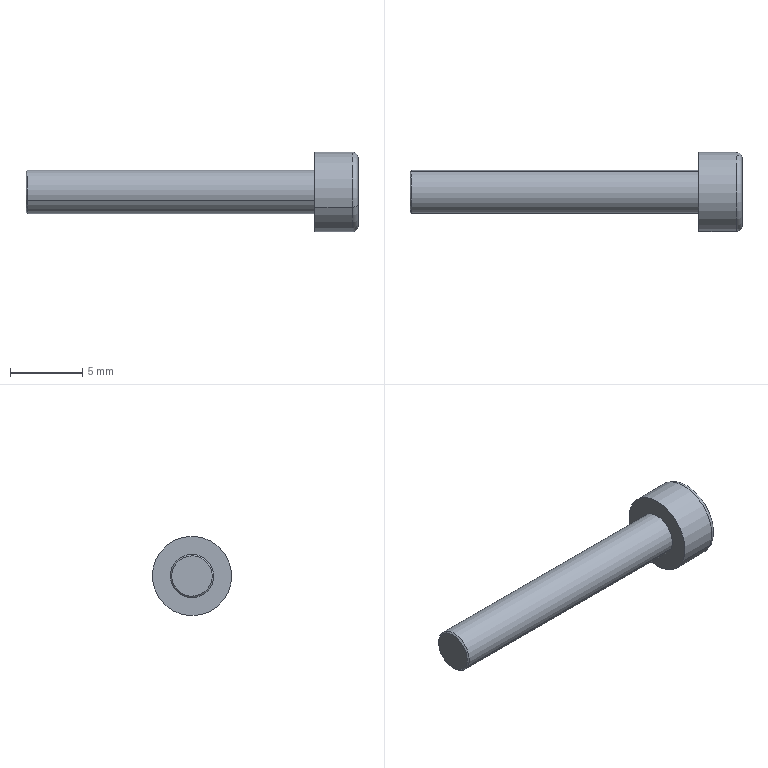Component | SolidWorks | hexagon socket head cap screws gb-1 | 1 solid | 25 faces | volume 204 mm3 | plane 15 | cone 4 | cylinder 4 | torus 2 | commonest cylinder face diameters 3 x2 5.5 x2